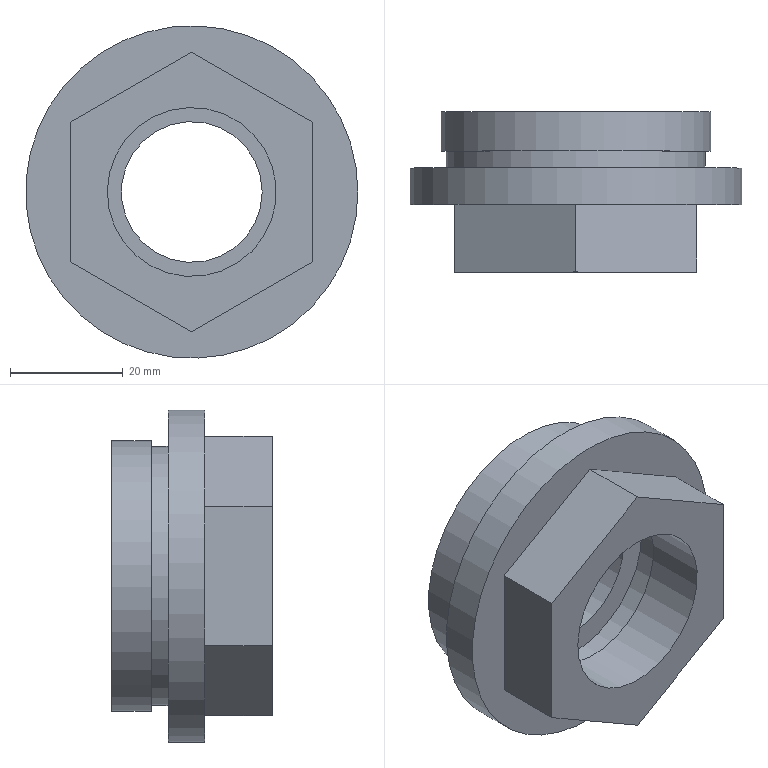Component | NX | VALVEBONNET | 1 solid | 21 faces | volume 32654 mm3 | plane 14 | cylinder 7 | commonest cylinder face diameters 48 x1 46 x1 59 x1 35 x1 30 x1 34 x1 25 x1